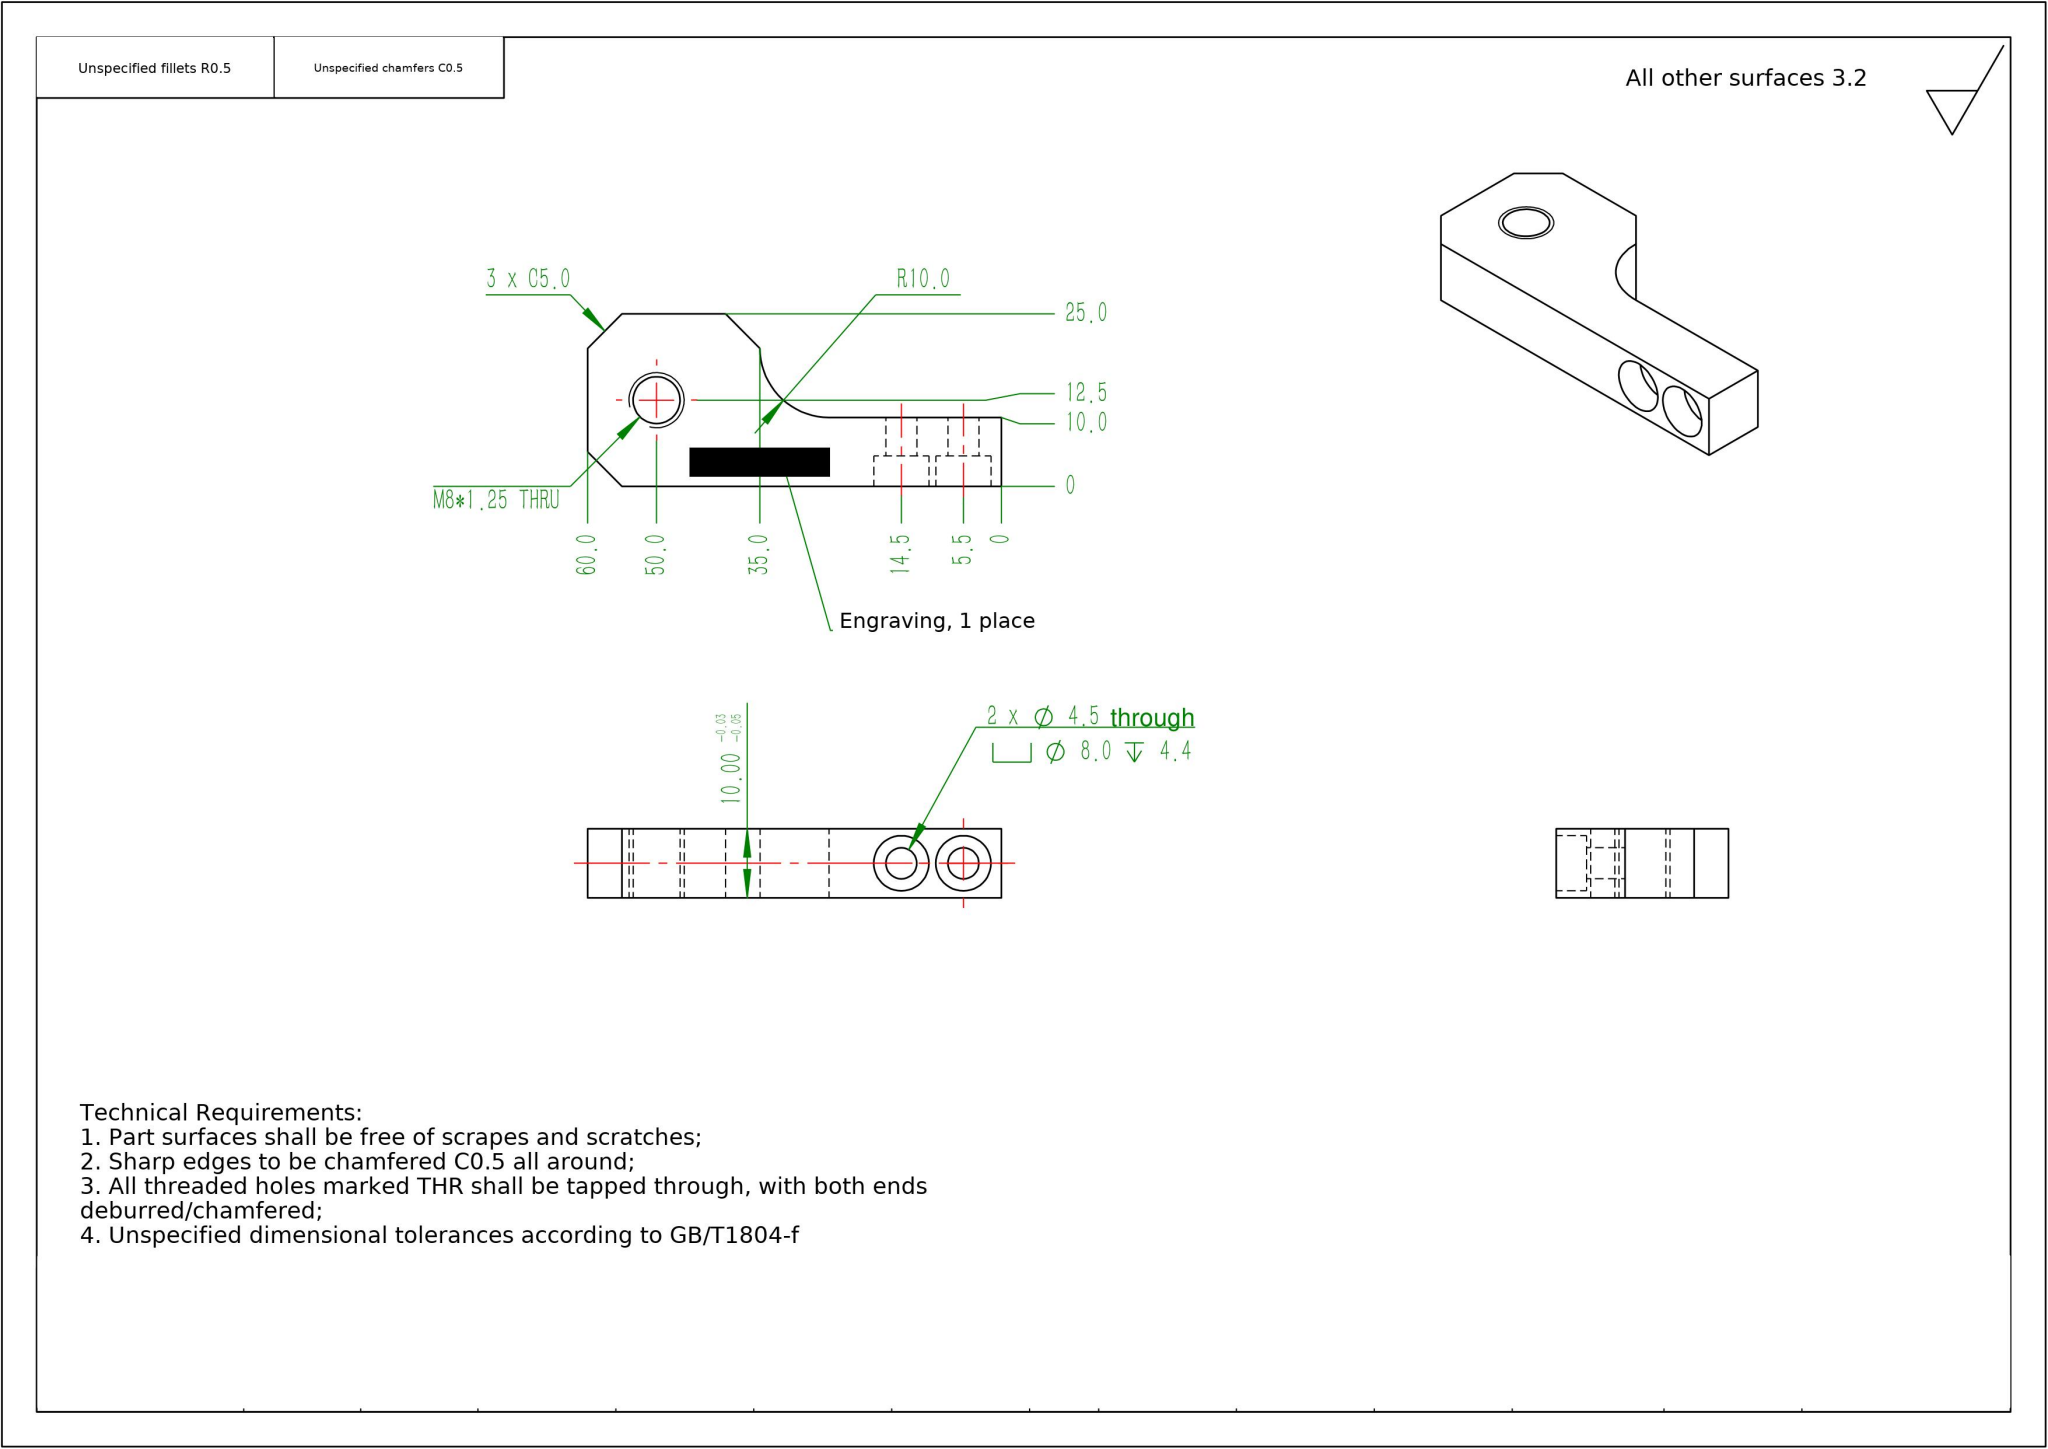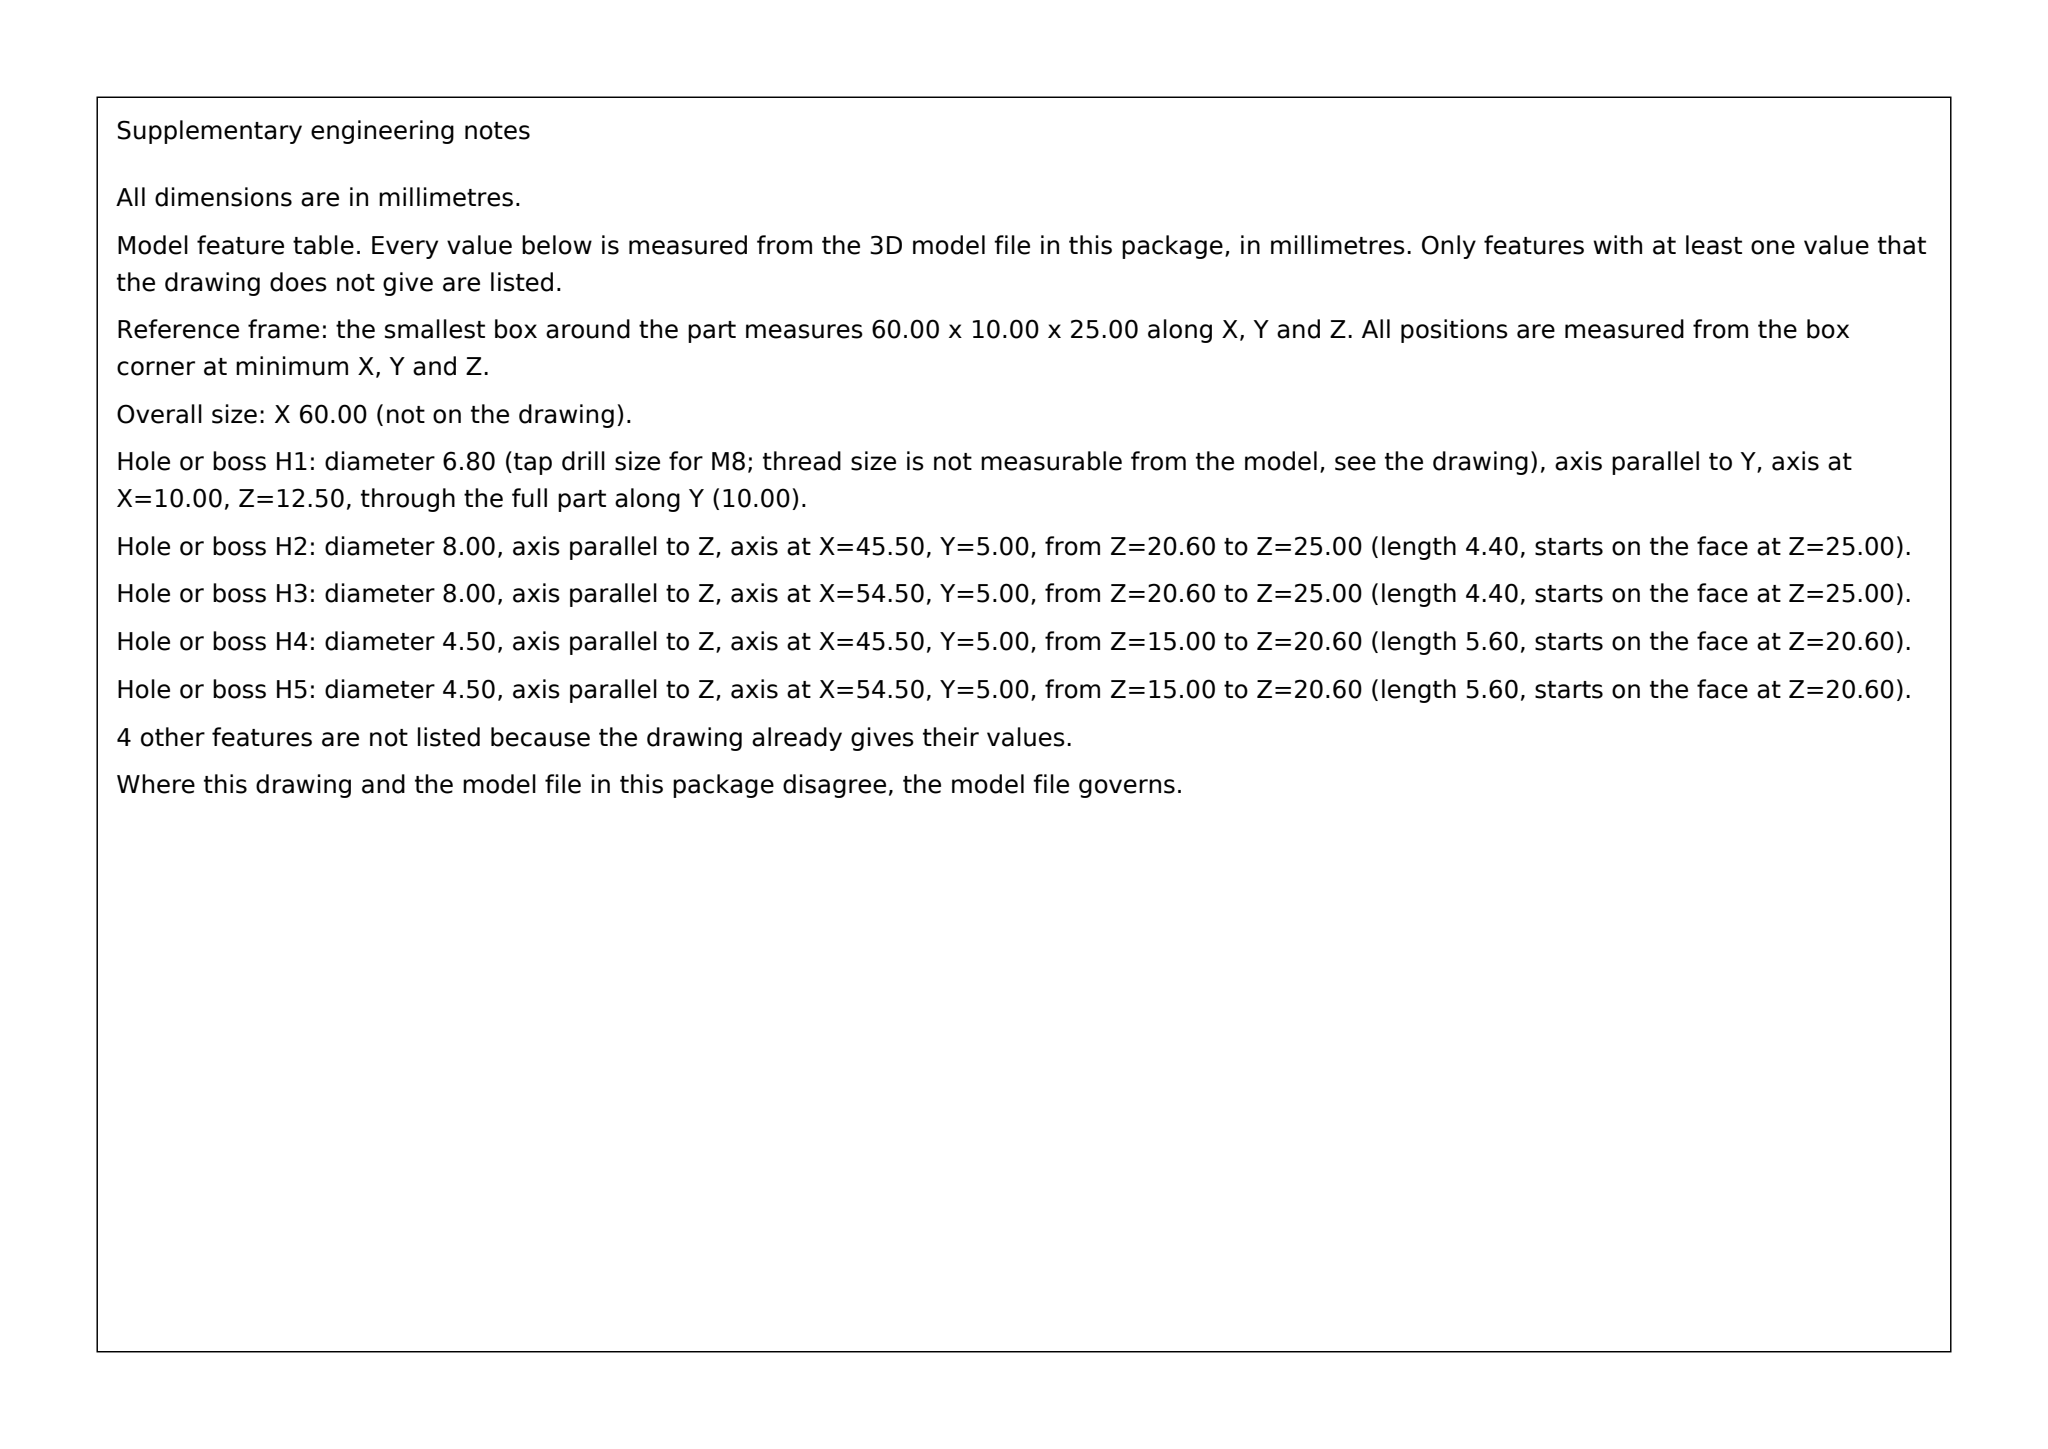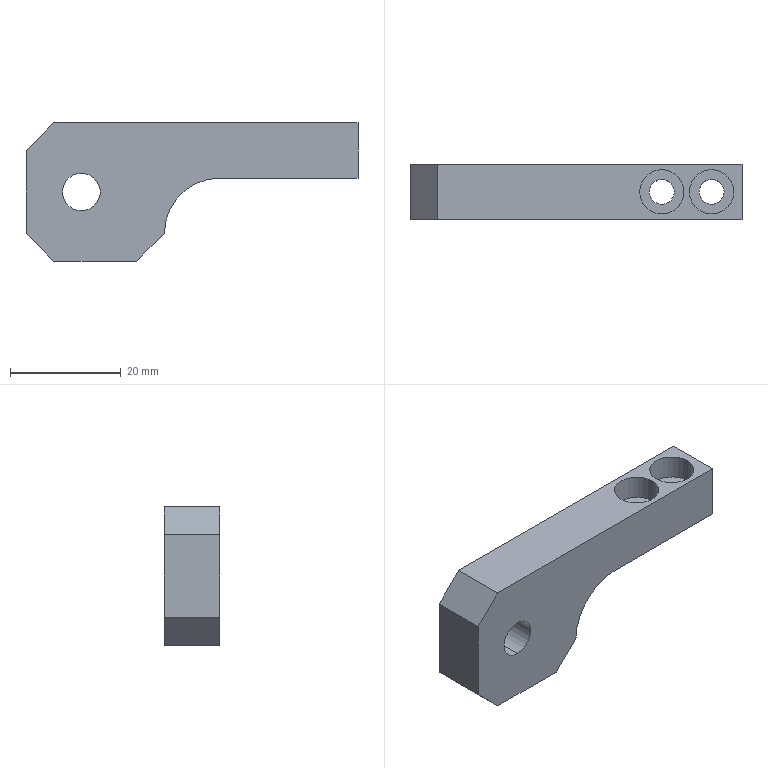Part | SolidWorks | mm | 1 solid | 23 faces | box 60 x 10 x 25 mm | volume 8606 mm3 | plane 12 | cylinder 11 | commonest cylinder face diameters 8 x4 4.5 x4 6.8 x2 20 x1
STEP:
#1=CARTESIAN_POINT('',(10.,0.,9.1));
#2=VERTEX_POINT('',#1);
#3=CARTESIAN_POINT('',(10.,0.,15.9));
#4=VERTEX_POINT('',#3);
#5=CARTESIAN_POINT('',(10.,0.,12.5));
#6=DIRECTION('',(0.,1.,0.));
#7=DIRECTION('',(0.,0.,1.));
#8=AXIS2_PLACEMENT_3D('',#5,#6,#7);
#9=CIRCLE('',#8,3.4);
#10=EDGE_CURVE('',#2,#4,#9,.T.);
#11=ORIENTED_EDGE('',*,*,#10,.F.);
#12=CARTESIAN_POINT('',(10.,10.,9.1));
#13=VERTEX_POINT('',#12);
#14=CARTESIAN_POINT('',(10.,10.,9.1));
#15=DIRECTION('',(0.,1.,0.));
#16=VECTOR('',#15,1000.);
#17=LINE('',#14,#16);
#18=EDGE_CURVE('',#2,#13,#17,.T.);
#19=ORIENTED_EDGE('',*,*,#18,.T.);
#20=CARTESIAN_POINT('',(10.,10.,15.9));
#21=VERTEX_POINT('',#20);
#22=CARTESIAN_POINT('',(10.,10.,12.5));
#23=DIRECTION('',(0.,1.,0.));
#24=DIRECTION('',(0.,0.,1.));
#25=AXIS2_PLACEMENT_3D('',#22,#23,#24);
#26=CIRCLE('',#25,3.4);
#27=EDGE_CURVE('',#13,#21,#26,.T.);
#28=ORIENTED_EDGE('',*,*,#27,.T.);
#29=CARTESIAN_POINT('',(10.,10.,15.9));
#30=DIRECTION('',(0.,1.,0.));
#31=VECTOR('',#30,1000.);
#32=LINE('',#29,#31);
#33=EDGE_CURVE('',#4,#21,#32,.T.);
#34=ORIENTED_EDGE('',*,*,#33,.F.);
#35=EDGE_LOOP('',(#11,#19,#28,#34));
#36=FACE_OUTER_BOUND('',#35,.T.);
#37=CARTESIAN_POINT('',(10.,10.,12.5));
#38=DIRECTION('',(0.,1.,0.));
#39=DIRECTION('',(0.,0.,1.));
#40=AXIS2_PLACEMENT_3D('',#37,#38,#39);
#41=CYLINDRICAL_SURFACE('',#40,3.4);
#42=ADVANCED_FACE('',(#36),#41,.F.);
#43=CARTESIAN_POINT('',(41.5,5.,20.6));
#44=VERTEX_POINT('',#43);
#45=CARTESIAN_POINT('',(49.5,5.,20.6));
#46=VERTEX_POINT('',#45);
#47=CARTESIAN_POINT('',(45.5,5.,20.6));
#48=DIRECTION('',(0.,0.,1.));
#49=DIRECTION('',(1.,0.,0.));
#50=AXIS2_PLACEMENT_3D('',#47,#48,#49);
#51=CIRCLE('',#50,4.);
#52=EDGE_CURVE('',#44,#46,#51,.T.);
#53=ORIENTED_EDGE('',*,*,#52,.F.);
#54=CARTESIAN_POINT('',(41.5,5.,25.));
#55=VERTEX_POINT('',#54);
#56=CARTESIAN_POINT('',(41.5,5.,25.));
#57=DIRECTION('',(0.,0.,1.));
#58=VECTOR('',#57,1000.);
#59=LINE('',#56,#58);
#60=EDGE_CURVE('',#44,#55,#59,.T.);
#61=ORIENTED_EDGE('',*,*,#60,.T.);
#62=CARTESIAN_POINT('',(49.5,5.,25.));
#63=VERTEX_POINT('',#62);
#64=CARTESIAN_POINT('',(45.5,5.,25.));
#65=DIRECTION('',(0.,0.,1.));
#66=DIRECTION('',(1.,0.,0.));
#67=AXIS2_PLACEMENT_3D('',#64,#65,#66);
#68=CIRCLE('',#67,4.);
#69=EDGE_CURVE('',#55,#63,#68,.T.);
#70=ORIENTED_EDGE('',*,*,#69,.T.);
#71=CARTESIAN_POINT('',(49.5,5.,25.));
#72=DIRECTION('',(0.,0.,1.));
#73=VECTOR('',#72,1000.);
#74=LINE('',#71,#73);
#75=EDGE_CURVE('',#46,#63,#74,.T.);
#76=ORIENTED_EDGE('',*,*,#75,.F.);
#77=EDGE_LOOP('',(#53,#61,#70,#76));
#78=FACE_OUTER_BOUND('',#77,.T.);
#79=CARTESIAN_POINT('',(45.5,5.,25.));
#80=DIRECTION('',(0.,0.,1.));
#81=DIRECTION('',(1.,0.,0.));
#82=AXIS2_PLACEMENT_3D('',#79,#80,#81);
#83=CYLINDRICAL_SURFACE('',#82,4.);
#84=ADVANCED_FACE('',(#78),#83,.F.);
#85=CARTESIAN_POINT('',(43.25,5.,15.));
#86=VERTEX_POINT('',#85);
#87=CARTESIAN_POINT('',(47.75,5.,15.));
#88=VERTEX_POINT('',#87);
#89=CARTESIAN_POINT('',(45.5,5.,15.));
#90=DIRECTION('',(0.,0.,1.));
#91=DIRECTION('',(1.,0.,0.));
#92=AXIS2_PLACEMENT_3D('',#89,#90,#91);
#93=CIRCLE('',#92,2.25);
#94=EDGE_CURVE('',#86,#88,#93,.T.);
#95=ORIENTED_EDGE('',*,*,#94,.F.);
#96=CARTESIAN_POINT('',(43.25,5.,20.6));
#97=VERTEX_POINT('',#96);
#98=CARTESIAN_POINT('',(43.25,5.,25.));
#99=DIRECTION('',(0.,0.,1.));
#100=VECTOR('',#99,1000.);
#101=LINE('',#98,#100);
#102=EDGE_CURVE('',#86,#97,#101,.T.);
#103=ORIENTED_EDGE('',*,*,#102,.T.);
#104=CARTESIAN_POINT('',(47.75,5.,20.6));
#105=VERTEX_POINT('',#104);
#106=CARTESIAN_POINT('',(45.5,5.,20.6));
#107=DIRECTION('',(0.,0.,1.));
#108=DIRECTION('',(1.,0.,0.));
#109=AXIS2_PLACEMENT_3D('',#106,#107,#108);
#110=CIRCLE('',#109,2.25);
#111=EDGE_CURVE('',#97,#105,#110,.T.);
#112=ORIENTED_EDGE('',*,*,#111,.T.);
#113=CARTESIAN_POINT('',(47.75,5.,25.));
#114=DIRECTION('',(0.,0.,1.));
#115=VECTOR('',#114,1000.);
#116=LINE('',#113,#115);
#117=EDGE_CURVE('',#88,#105,#116,.T.);
#118=ORIENTED_EDGE('',*,*,#117,.F.);
#119=EDGE_LOOP('',(#95,#103,#112,#118));
#120=FACE_OUTER_BOUND('',#119,.T.);
#121=CARTESIAN_POINT('',(45.5,5.,25.));
#122=DIRECTION('',(0.,0.,1.));
#123=DIRECTION('',(1.,0.,0.));
#124=AXIS2_PLACEMENT_3D('',#121,#122,#123);
#125=CYLINDRICAL_SURFACE('',#124,2.25);
#126=ADVANCED_FACE('',(#120),#125,.F.);
#127=CARTESIAN_POINT('',(50.5,5.,20.6));
#128=VERTEX_POINT('',#127);
#129=CARTESIAN_POINT('',(58.5,5.,20.6));
#130=VERTEX_POINT('',#129);
#131=CARTESIAN_POINT('',(54.5,5.,20.6));
#132=DIRECTION('',(0.,0.,1.));
#133=DIRECTION('',(1.,0.,0.));
#134=AXIS2_PLACEMENT_3D('',#131,#132,#133);
#135=CIRCLE('',#134,4.);
#136=EDGE_CURVE('',#128,#130,#135,.T.);
#137=ORIENTED_EDGE('',*,*,#136,.F.);
#138=CARTESIAN_POINT('',(50.5,5.,25.));
#139=VERTEX_POINT('',#138);
#140=CARTESIAN_POINT('',(50.5,5.,25.));
#141=DIRECTION('',(0.,0.,1.));
#142=VECTOR('',#141,1000.);
#143=LINE('',#140,#142);
#144=EDGE_CURVE('',#128,#139,#143,.T.);
#145=ORIENTED_EDGE('',*,*,#144,.T.);
#146=CARTESIAN_POINT('',(58.5,5.,25.));
#147=VERTEX_POINT('',#146);
#148=CARTESIAN_POINT('',(54.5,5.,25.));
#149=DIRECTION('',(0.,0.,1.));
#150=DIRECTION('',(1.,0.,0.));
#151=AXIS2_PLACEMENT_3D('',#148,#149,#150);
#152=CIRCLE('',#151,4.);
#153=EDGE_CURVE('',#139,#147,#152,.T.);
#154=ORIENTED_EDGE('',*,*,#153,.T.);
#155=CARTESIAN_POINT('',(58.5,5.,25.));
#156=DIRECTION('',(0.,0.,1.));
#157=VECTOR('',#156,1000.);
#158=LINE('',#155,#157);
#159=EDGE_CURVE('',#130,#147,#158,.T.);
#160=ORIENTED_EDGE('',*,*,#159,.F.);
#161=EDGE_LOOP('',(#137,#145,#154,#160));
#162=FACE_OUTER_BOUND('',#161,.T.);
#163=CARTESIAN_POINT('',(54.5,5.,25.));
#164=DIRECTION('',(0.,0.,1.));
#165=DIRECTION('',(1.,0.,0.));
#166=AXIS2_PLACEMENT_3D('',#163,#164,#165);
#167=CYLINDRICAL_SURFACE('',#166,4.);
#168=ADVANCED_FACE('',(#162),#167,.F.);
#169=CARTESIAN_POINT('',(52.25,5.,15.));
#170=VERTEX_POINT('',#169);
#171=CARTESIAN_POINT('',(56.75,5.,15.));
#172=VERTEX_POINT('',#171);
#173=CARTESIAN_POINT('',(54.5,5.,15.));
#174=DIRECTION('',(0.,0.,1.));
#175=DIRECTION('',(1.,0.,0.));
#176=AXIS2_PLACEMENT_3D('',#173,#174,#175);
#177=CIRCLE('',#176,2.25);
#178=EDGE_CURVE('',#170,#172,#177,.T.);
#179=ORIENTED_EDGE('',*,*,#178,.F.);
#180=CARTESIAN_POINT('',(52.25,5.,20.6));
#181=VERTEX_POINT('',#180);
#182=CARTESIAN_POINT('',(52.25,5.,25.));
#183=DIRECTION('',(0.,0.,1.));
#184=VECTOR('',#183,1000.);
#185=LINE('',#182,#184);
#186=EDGE_CURVE('',#170,#181,#185,.T.);
#187=ORIENTED_EDGE('',*,*,#186,.T.);
#188=CARTESIAN_POINT('',(56.75,5.,20.6));
#189=VERTEX_POINT('',#188);
#190=CARTESIAN_POINT('',(54.5,5.,20.6));
#191=DIRECTION('',(0.,0.,1.));
#192=DIRECTION('',(1.,0.,0.));
#193=AXIS2_PLACEMENT_3D('',#190,#191,#192);
#194=CIRCLE('',#193,2.25);
#195=EDGE_CURVE('',#181,#189,#194,.T.);
#196=ORIENTED_EDGE('',*,*,#195,.T.);
#197=CARTESIAN_POINT('',(56.75,5.,25.));
#198=DIRECTION('',(0.,0.,1.));
#199=VECTOR('',#198,1000.);
#200=LINE('',#197,#199);
#201=EDGE_CURVE('',#172,#189,#200,.T.);
#202=ORIENTED_EDGE('',*,*,#201,.F.);
#203=EDGE_LOOP('',(#179,#187,#196,#202));
#204=FACE_OUTER_BOUND('',#203,.T.);
#205=CARTESIAN_POINT('',(54.5,5.,25.));
#206=DIRECTION('',(0.,0.,1.));
#207=DIRECTION('',(1.,0.,0.));
#208=AXIS2_PLACEMENT_3D('',#205,#206,#207);
#209=CYLINDRICAL_SURFACE('',#208,2.25);
#210=ADVANCED_FACE('',(#204),#209,.F.);
#211=CARTESIAN_POINT('',(5.,0.,-0.));
#212=VERTEX_POINT('',#211);
#213=CARTESIAN_POINT('',(20.,0.,-0.));
#214=VERTEX_POINT('',#213);
#215=CARTESIAN_POINT('',(0.,0.,0.));
#216=DIRECTION('',(1.,0.,-0.));
#217=VECTOR('',#216,1000.);
#218=LINE('',#215,#217);
#219=EDGE_CURVE('',#212,#214,#218,.T.);
#220=ORIENTED_EDGE('',*,*,#219,.F.);
#221=CARTESIAN_POINT('',(5.,10.,-0.));
#222=VERTEX_POINT('',#221);
#223=CARTESIAN_POINT('',(5.,10.,-0.));
#224=DIRECTION('',(0.,1.,0.));
#225=VECTOR('',#224,1000.);
#226=LINE('',#223,#225);
#227=EDGE_CURVE('',#212,#222,#226,.T.);
#228=ORIENTED_EDGE('',*,*,#227,.T.);
#229=CARTESIAN_POINT('',(20.,10.,-0.));
#230=VERTEX_POINT('',#229);
#231=CARTESIAN_POINT('',(0.,10.,0.));
#232=DIRECTION('',(1.,0.,-0.));
#233=VECTOR('',#232,1000.);
#234=LINE('',#231,#233);
#235=EDGE_CURVE('',#222,#230,#234,.T.);
#236=ORIENTED_EDGE('',*,*,#235,.T.);
#237=CARTESIAN_POINT('',(20.,10.,-0.));
#238=DIRECTION('',(0.,-1.,0.));
#239=VECTOR('',#238,1000.);
#240=LINE('',#237,#239);
#241=EDGE_CURVE('',#230,#214,#240,.T.);
#242=ORIENTED_EDGE('',*,*,#241,.T.);
#243=EDGE_LOOP('',(#220,#228,#236,#242));
#244=FACE_OUTER_BOUND('',#243,.T.);
#245=CARTESIAN_POINT('',(0.,10.,0.));
#246=DIRECTION('',(-0.,0.,-1.));
#247=DIRECTION('',(-1.,0.,0.));
#248=AXIS2_PLACEMENT_3D('',#245,#246,#247);
#249=PLANE('',#248);
#250=ADVANCED_FACE('',(#244),#249,.T.);
#251=CARTESIAN_POINT('',(0.,0.,5.));
#252=VERTEX_POINT('',#251);
#253=CARTESIAN_POINT('',(0.,0.,20.));
#254=VERTEX_POINT('',#253);
#255=CARTESIAN_POINT('',(0.,0.,0.));
#256=DIRECTION('',(0.,0.,1.));
#257=VECTOR('',#256,1000.);
#258=LINE('',#255,#257);
#259=EDGE_CURVE('',#252,#254,#258,.T.);
#260=ORIENTED_EDGE('',*,*,#259,.T.);
#261=CARTESIAN_POINT('',(0.,10.,20.));
#262=VERTEX_POINT('',#261);
#263=CARTESIAN_POINT('',(0.,10.,20.));
#264=DIRECTION('',(0.,1.,0.));
#265=VECTOR('',#264,1000.);
#266=LINE('',#263,#265);
#267=EDGE_CURVE('',#254,#262,#266,.T.);
#268=ORIENTED_EDGE('',*,*,#267,.T.);
#269=CARTESIAN_POINT('',(0.,10.,5.));
#270=VERTEX_POINT('',#269);
#271=CARTESIAN_POINT('',(0.,10.,0.));
#272=DIRECTION('',(0.,0.,1.));
#273=VECTOR('',#272,1000.);
#274=LINE('',#271,#273);
#275=EDGE_CURVE('',#270,#262,#274,.T.);
#276=ORIENTED_EDGE('',*,*,#275,.F.);
#277=CARTESIAN_POINT('',(0.,0.,5.));
#278=DIRECTION('',(0.,-1.,0.));
#279=VECTOR('',#278,1000.);
#280=LINE('',#277,#279);
#281=EDGE_CURVE('',#270,#252,#280,.T.);
#282=ORIENTED_EDGE('',*,*,#281,.T.);
#283=EDGE_LOOP('',(#260,#268,#276,#282));
#284=FACE_OUTER_BOUND('',#283,.T.);
#285=CARTESIAN_POINT('',(0.,10.,0.));
#286=DIRECTION('',(1.,0.,-0.));
#287=DIRECTION('',(-0.,0.,-1.));
#288=AXIS2_PLACEMENT_3D('',#285,#286,#287);
#289=PLANE('',#288);
#290=ADVANCED_FACE('',(#284),#289,.F.);
#291=CARTESIAN_POINT('',(45.5,5.,25.));
#292=DIRECTION('',(0.,0.,1.));
#293=DIRECTION('',(1.,0.,0.));
#294=AXIS2_PLACEMENT_3D('',#291,#292,#293);
#295=CIRCLE('',#294,4.);
#296=EDGE_CURVE('',#63,#55,#295,.T.);
#297=ORIENTED_EDGE('',*,*,#296,.F.);
#298=ORIENTED_EDGE('',*,*,#69,.F.);
#299=EDGE_LOOP('',(#297,#298));
#300=FACE_BOUND('',#299,.T.);
#301=CARTESIAN_POINT('',(54.5,5.,25.));
#302=DIRECTION('',(0.,0.,1.));
#303=DIRECTION('',(1.,0.,0.));
#304=AXIS2_PLACEMENT_3D('',#301,#302,#303);
#305=CIRCLE('',#304,4.);
#306=EDGE_CURVE('',#147,#139,#305,.T.);
#307=ORIENTED_EDGE('',*,*,#306,.F.);
#308=ORIENTED_EDGE('',*,*,#153,.F.);
#309=EDGE_LOOP('',(#307,#308));
#310=FACE_BOUND('',#309,.T.);
#311=CARTESIAN_POINT('',(5.,10.,25.));
#312=VERTEX_POINT('',#311);
#313=CARTESIAN_POINT('',(60.,10.,25.));
#314=VERTEX_POINT('',#313);
#315=CARTESIAN_POINT('',(-0.,10.,25.));
#316=DIRECTION('',(1.,0.,0.));
#317=VECTOR('',#316,1000.);
#318=LINE('',#315,#317);
#319=EDGE_CURVE('',#312,#314,#318,.T.);
#320=ORIENTED_EDGE('',*,*,#319,.F.);
#321=CARTESIAN_POINT('',(5.,0.,25.));
#322=VERTEX_POINT('',#321);
#323=CARTESIAN_POINT('',(5.,10.,25.));
#324=DIRECTION('',(0.,-1.,0.));
#325=VECTOR('',#324,1000.);
#326=LINE('',#323,#325);
#327=EDGE_CURVE('',#312,#322,#326,.T.);
#328=ORIENTED_EDGE('',*,*,#327,.T.);
#329=CARTESIAN_POINT('',(60.,0.,25.));
#330=VERTEX_POINT('',#329);
#331=CARTESIAN_POINT('',(-0.,0.,25.));
#332=DIRECTION('',(1.,0.,0.));
#333=VECTOR('',#332,1000.);
#334=LINE('',#331,#333);
#335=EDGE_CURVE('',#322,#330,#334,.T.);
#336=ORIENTED_EDGE('',*,*,#335,.T.);
#337=CARTESIAN_POINT('',(60.,10.,25.));
#338=DIRECTION('',(0.,-1.,0.));
#339=VECTOR('',#338,1000.);
#340=LINE('',#337,#339);
#341=EDGE_CURVE('',#314,#330,#340,.T.);
#342=ORIENTED_EDGE('',*,*,#341,.F.);
#343=EDGE_LOOP('',(#320,#328,#336,#342));
#344=FACE_OUTER_BOUND('',#343,.T.);
#345=CARTESIAN_POINT('',(-0.,10.,25.));
#346=DIRECTION('',(0.,0.,-1.));
#347=DIRECTION('',(-1.,0.,-0.));
#348=AXIS2_PLACEMENT_3D('',#345,#346,#347);
#349=PLANE('',#348);
#350=ADVANCED_FACE('',(#300,#310,#344),#349,.F.);
#351=CARTESIAN_POINT('',(60.,0.,15.));
#352=VERTEX_POINT('',#351);
#353=CARTESIAN_POINT('',(60.,0.,-0.));
#354=DIRECTION('',(0.,0.,1.));
#355=VECTOR('',#354,1000.);
#356=LINE('',#353,#355);
#357=EDGE_CURVE('',#352,#330,#356,.T.);
#358=ORIENTED_EDGE('',*,*,#357,.F.);
#359=CARTESIAN_POINT('',(60.,10.,15.));
#360=VERTEX_POINT('',#359);
#361=CARTESIAN_POINT('',(60.,10.,15.));
#362=DIRECTION('',(0.,-1.,0.));
#363=VECTOR('',#362,1000.);
#364=LINE('',#361,#363);
#365=EDGE_CURVE('',#360,#352,#364,.T.);
#366=ORIENTED_EDGE('',*,*,#365,.F.);
#367=CARTESIAN_POINT('',(60.,10.,-0.));
#368=DIRECTION('',(0.,0.,1.));
#369=VECTOR('',#368,1000.);
#370=LINE('',#367,#369);
#371=EDGE_CURVE('',#360,#314,#370,.T.);
#372=ORIENTED_EDGE('',*,*,#371,.T.);
#373=ORIENTED_EDGE('',*,*,#341,.T.);
#374=EDGE_LOOP('',(#358,#366,#372,#373));
#375=FACE_OUTER_BOUND('',#374,.T.);
#376=CARTESIAN_POINT('',(60.,10.,-0.));
#377=DIRECTION('',(1.,0.,-0.));
#378=DIRECTION('',(-0.,0.,-1.));
#379=AXIS2_PLACEMENT_3D('',#376,#377,#378);
#380=PLANE('',#379);
#381=ADVANCED_FACE('',(#375),#380,.T.);
#382=CARTESIAN_POINT('',(45.5,5.,15.));
#383=DIRECTION('',(0.,0.,1.));
#384=DIRECTION('',(1.,0.,0.));
#385=AXIS2_PLACEMENT_3D('',#382,#383,#384);
#386=CIRCLE('',#385,2.25);
#387=EDGE_CURVE('',#88,#86,#386,.T.);
#388=ORIENTED_EDGE('',*,*,#387,.T.);
#389=ORIENTED_EDGE('',*,*,#94,.T.);
#390=EDGE_LOOP('',(#388,#389));
#391=FACE_BOUND('',#390,.T.);
#392=CARTESIAN_POINT('',(54.5,5.,15.));
#393=DIRECTION('',(0.,0.,1.));
#394=DIRECTION('',(1.,0.,0.));
#395=AXIS2_PLACEMENT_3D('',#392,#393,#394);
#396=CIRCLE('',#395,2.25);
#397=EDGE_CURVE('',#172,#170,#396,.T.);
#398=ORIENTED_EDGE('',*,*,#397,.T.);
#399=ORIENTED_EDGE('',*,*,#178,.T.);
#400=EDGE_LOOP('',(#398,#399));
#401=FACE_BOUND('',#400,.T.);
#402=CARTESIAN_POINT('',(35.,0.,15.));
#403=VERTEX_POINT('',#402);
#404=CARTESIAN_POINT('',(0.,0.,15.));
#405=DIRECTION('',(-1.,0.,0.));
#406=VECTOR('',#405,1000.);
#407=LINE('',#404,#406);
#408=EDGE_CURVE('',#352,#403,#407,.T.);
#409=ORIENTED_EDGE('',*,*,#408,.T.);
#410=CARTESIAN_POINT('',(35.,10.,15.));
#411=VERTEX_POINT('',#410);
#412=CARTESIAN_POINT('',(35.,10.,15.));
#413=DIRECTION('',(0.,1.,0.));
#414=VECTOR('',#413,1000.);
#415=LINE('',#412,#414);
#416=EDGE_CURVE('',#403,#411,#415,.T.);
#417=ORIENTED_EDGE('',*,*,#416,.T.);
#418=CARTESIAN_POINT('',(0.,10.,15.));
#419=DIRECTION('',(-1.,0.,0.));
#420=VECTOR('',#419,1000.);
#421=LINE('',#418,#420);
#422=EDGE_CURVE('',#360,#411,#421,.T.);
#423=ORIENTED_EDGE('',*,*,#422,.F.);
#424=ORIENTED_EDGE('',*,*,#365,.T.);
#425=EDGE_LOOP('',(#409,#417,#423,#424));
#426=FACE_OUTER_BOUND('',#425,.T.);
#427=CARTESIAN_POINT('',(0.,10.,15.));
#428=DIRECTION('',(0.,0.,1.));
#429=DIRECTION('',(1.,0.,-0.));
#430=AXIS2_PLACEMENT_3D('',#427,#428,#429);
#431=PLANE('',#430);
#432=ADVANCED_FACE('',(#391,#401,#426),#431,.F.);
#433=CARTESIAN_POINT('',(10.,10.,12.5));
#434=DIRECTION('',(0.,1.,0.));
#435=DIRECTION('',(0.,0.,1.));
#436=AXIS2_PLACEMENT_3D('',#433,#434,#435);
#437=CIRCLE('',#436,3.4);
#438=EDGE_CURVE('',#21,#13,#437,.T.);
#439=ORIENTED_EDGE('',*,*,#438,.F.);
#440=ORIENTED_EDGE('',*,*,#27,.F.);
#441=EDGE_LOOP('',(#439,#440));
#442=FACE_BOUND('',#441,.T.);
#443=ORIENTED_EDGE('',*,*,#275,.T.);
#444=CARTESIAN_POINT('',(-10.,10.,10.));
#445=DIRECTION('',(0.7071,0.,0.7071));
#446=VECTOR('',#445,1000.);
#447=LINE('',#444,#446);
#448=EDGE_CURVE('',#262,#312,#447,.T.);
#449=ORIENTED_EDGE('',*,*,#448,.T.);
#450=ORIENTED_EDGE('',*,*,#319,.T.);
#451=ORIENTED_EDGE('',*,*,#371,.F.);
#452=ORIENTED_EDGE('',*,*,#422,.T.);
#453=CARTESIAN_POINT('',(25.,10.,5.));
#454=VERTEX_POINT('',#453);
#455=CARTESIAN_POINT('',(35.,10.,5.));
#456=DIRECTION('',(0.,-1.,0.));
#457=DIRECTION('',(0.,0.,1.));
#458=AXIS2_PLACEMENT_3D('',#455,#456,#457);
#459=CIRCLE('',#458,10.);
#460=EDGE_CURVE('',#411,#454,#459,.T.);
#461=ORIENTED_EDGE('',*,*,#460,.T.);
#462=CARTESIAN_POINT('',(10.,10.,-10.));
#463=DIRECTION('',(-0.7071,0.,-0.7071));
#464=VECTOR('',#463,1000.);
#465=LINE('',#462,#464);
#466=EDGE_CURVE('',#454,#230,#465,.T.);
#467=ORIENTED_EDGE('',*,*,#466,.T.);
#468=ORIENTED_EDGE('',*,*,#235,.F.);
#469=CARTESIAN_POINT('',(2.5,10.,2.5));
#470=DIRECTION('',(-0.7071,0.,0.7071));
#471=VECTOR('',#470,1000.);
#472=LINE('',#469,#471);
#473=EDGE_CURVE('',#222,#270,#472,.T.);
#474=ORIENTED_EDGE('',*,*,#473,.T.);
#475=EDGE_LOOP('',(#443,#449,#450,#451,#452,#461,#467,#468,#474));
#476=FACE_OUTER_BOUND('',#475,.T.);
#477=CARTESIAN_POINT('',(0.,10.,0.));
#478=DIRECTION('',(0.,1.,0.));
#479=DIRECTION('',(0.,0.,1.));
#480=AXIS2_PLACEMENT_3D('',#477,#478,#479);
#481=PLANE('',#480);
#482=ADVANCED_FACE('',(#442,#476),#481,.T.);
#483=CARTESIAN_POINT('',(10.,0.,12.5));
#484=DIRECTION('',(0.,1.,0.));
#485=DIRECTION('',(0.,0.,1.));
#486=AXIS2_PLACEMENT_3D('',#483,#484,#485);
#487=CIRCLE('',#486,3.4);
#488=EDGE_CURVE('',#4,#2,#487,.T.);
#489=ORIENTED_EDGE('',*,*,#488,.T.);
#490=ORIENTED_EDGE('',*,*,#10,.T.);
#491=EDGE_LOOP('',(#489,#490));
#492=FACE_BOUND('',#491,.T.);
#493=ORIENTED_EDGE('',*,*,#335,.F.);
#494=CARTESIAN_POINT('',(5.,0.,25.));
#495=DIRECTION('',(-0.7071,0.,-0.7071));
#496=VECTOR('',#495,1000.);
#497=LINE('',#494,#496);
#498=EDGE_CURVE('',#322,#254,#497,.T.);
#499=ORIENTED_EDGE('',*,*,#498,.T.);
#500=ORIENTED_EDGE('',*,*,#259,.F.);
#501=CARTESIAN_POINT('',(0.,0.,5.));
#502=DIRECTION('',(0.7071,0.,-0.7071));
#503=VECTOR('',#502,1000.);
#504=LINE('',#501,#503);
#505=EDGE_CURVE('',#252,#212,#504,.T.);
#506=ORIENTED_EDGE('',*,*,#505,.T.);
#507=ORIENTED_EDGE('',*,*,#219,.T.);
#508=CARTESIAN_POINT('',(25.,0.,5.));
#509=VERTEX_POINT('',#508);
#510=CARTESIAN_POINT('',(20.,0.,-0.));
#511=DIRECTION('',(0.7071,0.,0.7071));
#512=VECTOR('',#511,1000.);
#513=LINE('',#510,#512);
#514=EDGE_CURVE('',#214,#509,#513,.T.);
#515=ORIENTED_EDGE('',*,*,#514,.T.);
#516=CARTESIAN_POINT('',(35.,0.,5.));
#517=DIRECTION('',(0.,1.,0.));
#518=DIRECTION('',(0.,0.,1.));
#519=AXIS2_PLACEMENT_3D('',#516,#517,#518);
#520=CIRCLE('',#519,10.);
#521=EDGE_CURVE('',#509,#403,#520,.T.);
#522=ORIENTED_EDGE('',*,*,#521,.T.);
#523=ORIENTED_EDGE('',*,*,#408,.F.);
#524=ORIENTED_EDGE('',*,*,#357,.T.);
#525=EDGE_LOOP('',(#493,#499,#500,#506,#507,#515,#522,#523,#524));
#526=FACE_OUTER_BOUND('',#525,.T.);
#527=CARTESIAN_POINT('',(0.,0.,0.));
#528=DIRECTION('',(0.,1.,0.));
#529=DIRECTION('',(0.,0.,1.));
#530=AXIS2_PLACEMENT_3D('',#527,#528,#529);
#531=PLANE('',#530);
#532=ADVANCED_FACE('',(#492,#526),#531,.F.);
#533=ORIENTED_EDGE('',*,*,#186,.F.);
#534=ORIENTED_EDGE('',*,*,#397,.F.);
#535=ORIENTED_EDGE('',*,*,#201,.T.);
#536=CARTESIAN_POINT('',(54.5,5.,20.6));
#537=DIRECTION('',(0.,0.,1.));
#538=DIRECTION('',(1.,0.,0.));
#539=AXIS2_PLACEMENT_3D('',#536,#537,#538);
#540=CIRCLE('',#539,2.25);
#541=EDGE_CURVE('',#189,#181,#540,.T.);
#542=ORIENTED_EDGE('',*,*,#541,.T.);
#543=EDGE_LOOP('',(#533,#534,#535,#542));
#544=FACE_OUTER_BOUND('',#543,.T.);
#545=CARTESIAN_POINT('',(54.5,5.,25.));
#546=DIRECTION('',(0.,0.,1.));
#547=DIRECTION('',(1.,0.,0.));
#548=AXIS2_PLACEMENT_3D('',#545,#546,#547);
#549=CYLINDRICAL_SURFACE('',#548,2.25);
#550=ADVANCED_FACE('',(#544),#549,.F.);
#551=ORIENTED_EDGE('',*,*,#541,.F.);
#552=ORIENTED_EDGE('',*,*,#195,.F.);
#553=EDGE_LOOP('',(#551,#552));
#554=FACE_BOUND('',#553,.T.);
#555=CARTESIAN_POINT('',(54.5,5.,20.6));
#556=DIRECTION('',(0.,0.,1.));
#557=DIRECTION('',(1.,0.,0.));
#558=AXIS2_PLACEMENT_3D('',#555,#556,#557);
#559=CIRCLE('',#558,4.);
#560=EDGE_CURVE('',#130,#128,#559,.T.);
#561=ORIENTED_EDGE('',*,*,#560,.T.);
#562=ORIENTED_EDGE('',*,*,#136,.T.);
#563=EDGE_LOOP('',(#561,#562));
#564=FACE_OUTER_BOUND('',#563,.T.);
#565=CARTESIAN_POINT('',(56.75,5.,20.6));
#566=DIRECTION('',(0.,0.,-1.));
#567=DIRECTION('',(-1.,0.,0.));
#568=AXIS2_PLACEMENT_3D('',#565,#566,#567);
#569=PLANE('',#568);
#570=ADVANCED_FACE('',(#554,#564),#569,.F.);
#571=ORIENTED_EDGE('',*,*,#144,.F.);
#572=ORIENTED_EDGE('',*,*,#560,.F.);
#573=ORIENTED_EDGE('',*,*,#159,.T.);
#574=ORIENTED_EDGE('',*,*,#306,.T.);
#575=EDGE_LOOP('',(#571,#572,#573,#574));
#576=FACE_OUTER_BOUND('',#575,.T.);
#577=CARTESIAN_POINT('',(54.5,5.,25.));
#578=DIRECTION('',(0.,0.,1.));
#579=DIRECTION('',(1.,0.,0.));
#580=AXIS2_PLACEMENT_3D('',#577,#578,#579);
#581=CYLINDRICAL_SURFACE('',#580,4.);
#582=ADVANCED_FACE('',(#576),#581,.F.);
#583=ORIENTED_EDGE('',*,*,#102,.F.);
#584=ORIENTED_EDGE('',*,*,#387,.F.);
#585=ORIENTED_EDGE('',*,*,#117,.T.);
#586=CARTESIAN_POINT('',(45.5,5.,20.6));
#587=DIRECTION('',(0.,0.,1.));
#588=DIRECTION('',(1.,0.,0.));
#589=AXIS2_PLACEMENT_3D('',#586,#587,#588);
#590=CIRCLE('',#589,2.25);
#591=EDGE_CURVE('',#105,#97,#590,.T.);
#592=ORIENTED_EDGE('',*,*,#591,.T.);
#593=EDGE_LOOP('',(#583,#584,#585,#592));
#594=FACE_OUTER_BOUND('',#593,.T.);
#595=CARTESIAN_POINT('',(45.5,5.,25.));
#596=DIRECTION('',(0.,0.,1.));
#597=DIRECTION('',(1.,0.,0.));
#598=AXIS2_PLACEMENT_3D('',#595,#596,#597);
#599=CYLINDRICAL_SURFACE('',#598,2.25);
#600=ADVANCED_FACE('',(#594),#599,.F.);
#601=ORIENTED_EDGE('',*,*,#591,.F.);
#602=ORIENTED_EDGE('',*,*,#111,.F.);
#603=EDGE_LOOP('',(#601,#602));
#604=FACE_BOUND('',#603,.T.);
#605=CARTESIAN_POINT('',(45.5,5.,20.6));
#606=DIRECTION('',(0.,0.,1.));
#607=DIRECTION('',(1.,0.,0.));
#608=AXIS2_PLACEMENT_3D('',#605,#606,#607);
#609=CIRCLE('',#608,4.);
#610=EDGE_CURVE('',#46,#44,#609,.T.);
#611=ORIENTED_EDGE('',*,*,#610,.T.);
#612=ORIENTED_EDGE('',*,*,#52,.T.);
#613=EDGE_LOOP('',(#611,#612));
#614=FACE_OUTER_BOUND('',#613,.T.);
#615=CARTESIAN_POINT('',(47.75,5.,20.6));
#616=DIRECTION('',(0.,0.,-1.));
#617=DIRECTION('',(-1.,0.,0.));
#618=AXIS2_PLACEMENT_3D('',#615,#616,#617);
#619=PLANE('',#618);
#620=ADVANCED_FACE('',(#604,#614),#619,.F.);
#621=ORIENTED_EDGE('',*,*,#60,.F.);
#622=ORIENTED_EDGE('',*,*,#610,.F.);
#623=ORIENTED_EDGE('',*,*,#75,.T.);
#624=ORIENTED_EDGE('',*,*,#296,.T.);
#625=EDGE_LOOP('',(#621,#622,#623,#624));
#626=FACE_OUTER_BOUND('',#625,.T.);
#627=CARTESIAN_POINT('',(45.5,5.,25.));
#628=DIRECTION('',(0.,0.,1.));
#629=DIRECTION('',(1.,0.,0.));
#630=AXIS2_PLACEMENT_3D('',#627,#628,#629);
#631=CYLINDRICAL_SURFACE('',#630,4.);
#632=ADVANCED_FACE('',(#626),#631,.F.);
#633=ORIENTED_EDGE('',*,*,#18,.F.);
#634=ORIENTED_EDGE('',*,*,#488,.F.);
#635=ORIENTED_EDGE('',*,*,#33,.T.);
#636=ORIENTED_EDGE('',*,*,#438,.T.);
#637=EDGE_LOOP('',(#633,#634,#635,#636));
#638=FACE_OUTER_BOUND('',#637,.T.);
#639=CARTESIAN_POINT('',(10.,10.,12.5));
#640=DIRECTION('',(0.,1.,0.));
#641=DIRECTION('',(0.,0.,1.));
#642=AXIS2_PLACEMENT_3D('',#639,#640,#641);
#643=CYLINDRICAL_SURFACE('',#642,3.4);
#644=ADVANCED_FACE('',(#638),#643,.F.);
#645=ORIENTED_EDGE('',*,*,#460,.F.);
#646=ORIENTED_EDGE('',*,*,#416,.F.);
#647=ORIENTED_EDGE('',*,*,#521,.F.);
#648=CARTESIAN_POINT('',(25.,10.,5.));
#649=DIRECTION('',(0.,-1.,0.));
#650=VECTOR('',#649,1000.);
#651=LINE('',#648,#650);
#652=EDGE_CURVE('',#454,#509,#651,.T.);
#653=ORIENTED_EDGE('',*,*,#652,.F.);
#654=EDGE_LOOP('',(#645,#646,#647,#653));
#655=FACE_OUTER_BOUND('',#654,.T.);
#656=CARTESIAN_POINT('',(35.,10.,5.));
#657=DIRECTION('',(0.,-1.,0.));
#658=DIRECTION('',(0.,0.,-1.));
#659=AXIS2_PLACEMENT_3D('',#656,#657,#658);
#660=CYLINDRICAL_SURFACE('',#659,10.);
#661=ADVANCED_FACE('',(#655),#660,.F.);
#662=ORIENTED_EDGE('',*,*,#448,.F.);
#663=ORIENTED_EDGE('',*,*,#267,.F.);
#664=ORIENTED_EDGE('',*,*,#498,.F.);
#665=ORIENTED_EDGE('',*,*,#327,.F.);
#666=EDGE_LOOP('',(#662,#663,#664,#665));
#667=FACE_OUTER_BOUND('',#666,.T.);
#668=CARTESIAN_POINT('',(5.,10.,25.));
#669=DIRECTION('',(0.7071,0.,-0.7071));
#670=DIRECTION('',(0.,-1.,0.));
#671=AXIS2_PLACEMENT_3D('',#668,#669,#670);
#672=PLANE('',#671);
#673=ADVANCED_FACE('',(#667),#672,.F.);
#674=ORIENTED_EDGE('',*,*,#473,.F.);
#675=ORIENTED_EDGE('',*,*,#227,.F.);
#676=ORIENTED_EDGE('',*,*,#505,.F.);
#677=ORIENTED_EDGE('',*,*,#281,.F.);
#678=EDGE_LOOP('',(#674,#675,#676,#677));
#679=FACE_OUTER_BOUND('',#678,.T.);
#680=CARTESIAN_POINT('',(0.,10.,5.));
#681=DIRECTION('',(-0.7071,0.,-0.7071));
#682=DIRECTION('',(0.,1.,0.));
#683=AXIS2_PLACEMENT_3D('',#680,#681,#682);
#684=PLANE('',#683);
#685=ADVANCED_FACE('',(#679),#684,.T.);
#686=ORIENTED_EDGE('',*,*,#466,.F.);
#687=ORIENTED_EDGE('',*,*,#652,.T.);
#688=ORIENTED_EDGE('',*,*,#514,.F.);
#689=ORIENTED_EDGE('',*,*,#241,.F.);
#690=EDGE_LOOP('',(#686,#687,#688,#689));
#691=FACE_OUTER_BOUND('',#690,.T.);
#692=CARTESIAN_POINT('',(20.,10.,-0.));
#693=DIRECTION('',(-0.7071,0.,0.7071));
#694=DIRECTION('',(0.,-1.,0.));
#695=AXIS2_PLACEMENT_3D('',#692,#693,#694);
#696=PLANE('',#695);
#697=ADVANCED_FACE('',(#691),#696,.F.);
#698=CLOSED_SHELL('',(#42,#84,#126,#168,#210,#250,#290,#350,#381,#432,#482,#532,#550,#570,#582,#600,#620,#632,#644,#661,#673,#685,#697));
#699=MANIFOLD_SOLID_BREP('',#698);
#700=CARTESIAN_POINT('',(0.,0.,0.));
#701=DIRECTION('',(0.,0.,1.));
#702=DIRECTION('',(1.,0.,0.));
#703=AXIS2_PLACEMENT_3D('',#700,#701,#702);
#704=(LENGTH_UNIT()NAMED_UNIT(*)SI_UNIT(.MILLI.,.METRE.));
#705=UNCERTAINTY_MEASURE_WITH_UNIT(LENGTH_MEASURE(0.00001),#704,'','');
#706=(NAMED_UNIT(*)PLANE_ANGLE_UNIT()SI_UNIT($,.RADIAN.));
#707=(NAMED_UNIT(*)SI_UNIT($,.STERADIAN.)SOLID_ANGLE_UNIT());
#708=(GEOMETRIC_REPRESENTATION_CONTEXT(3)GLOBAL_UNCERTAINTY_ASSIGNED_CONTEXT((#705))GLOBAL_UNIT_ASSIGNED_CONTEXT((#704,#706,#707))REPRESENTATION_CONTEXT('',''));
#709=ADVANCED_BREP_SHAPE_REPRESENTATION('',(#699,#703),#708);